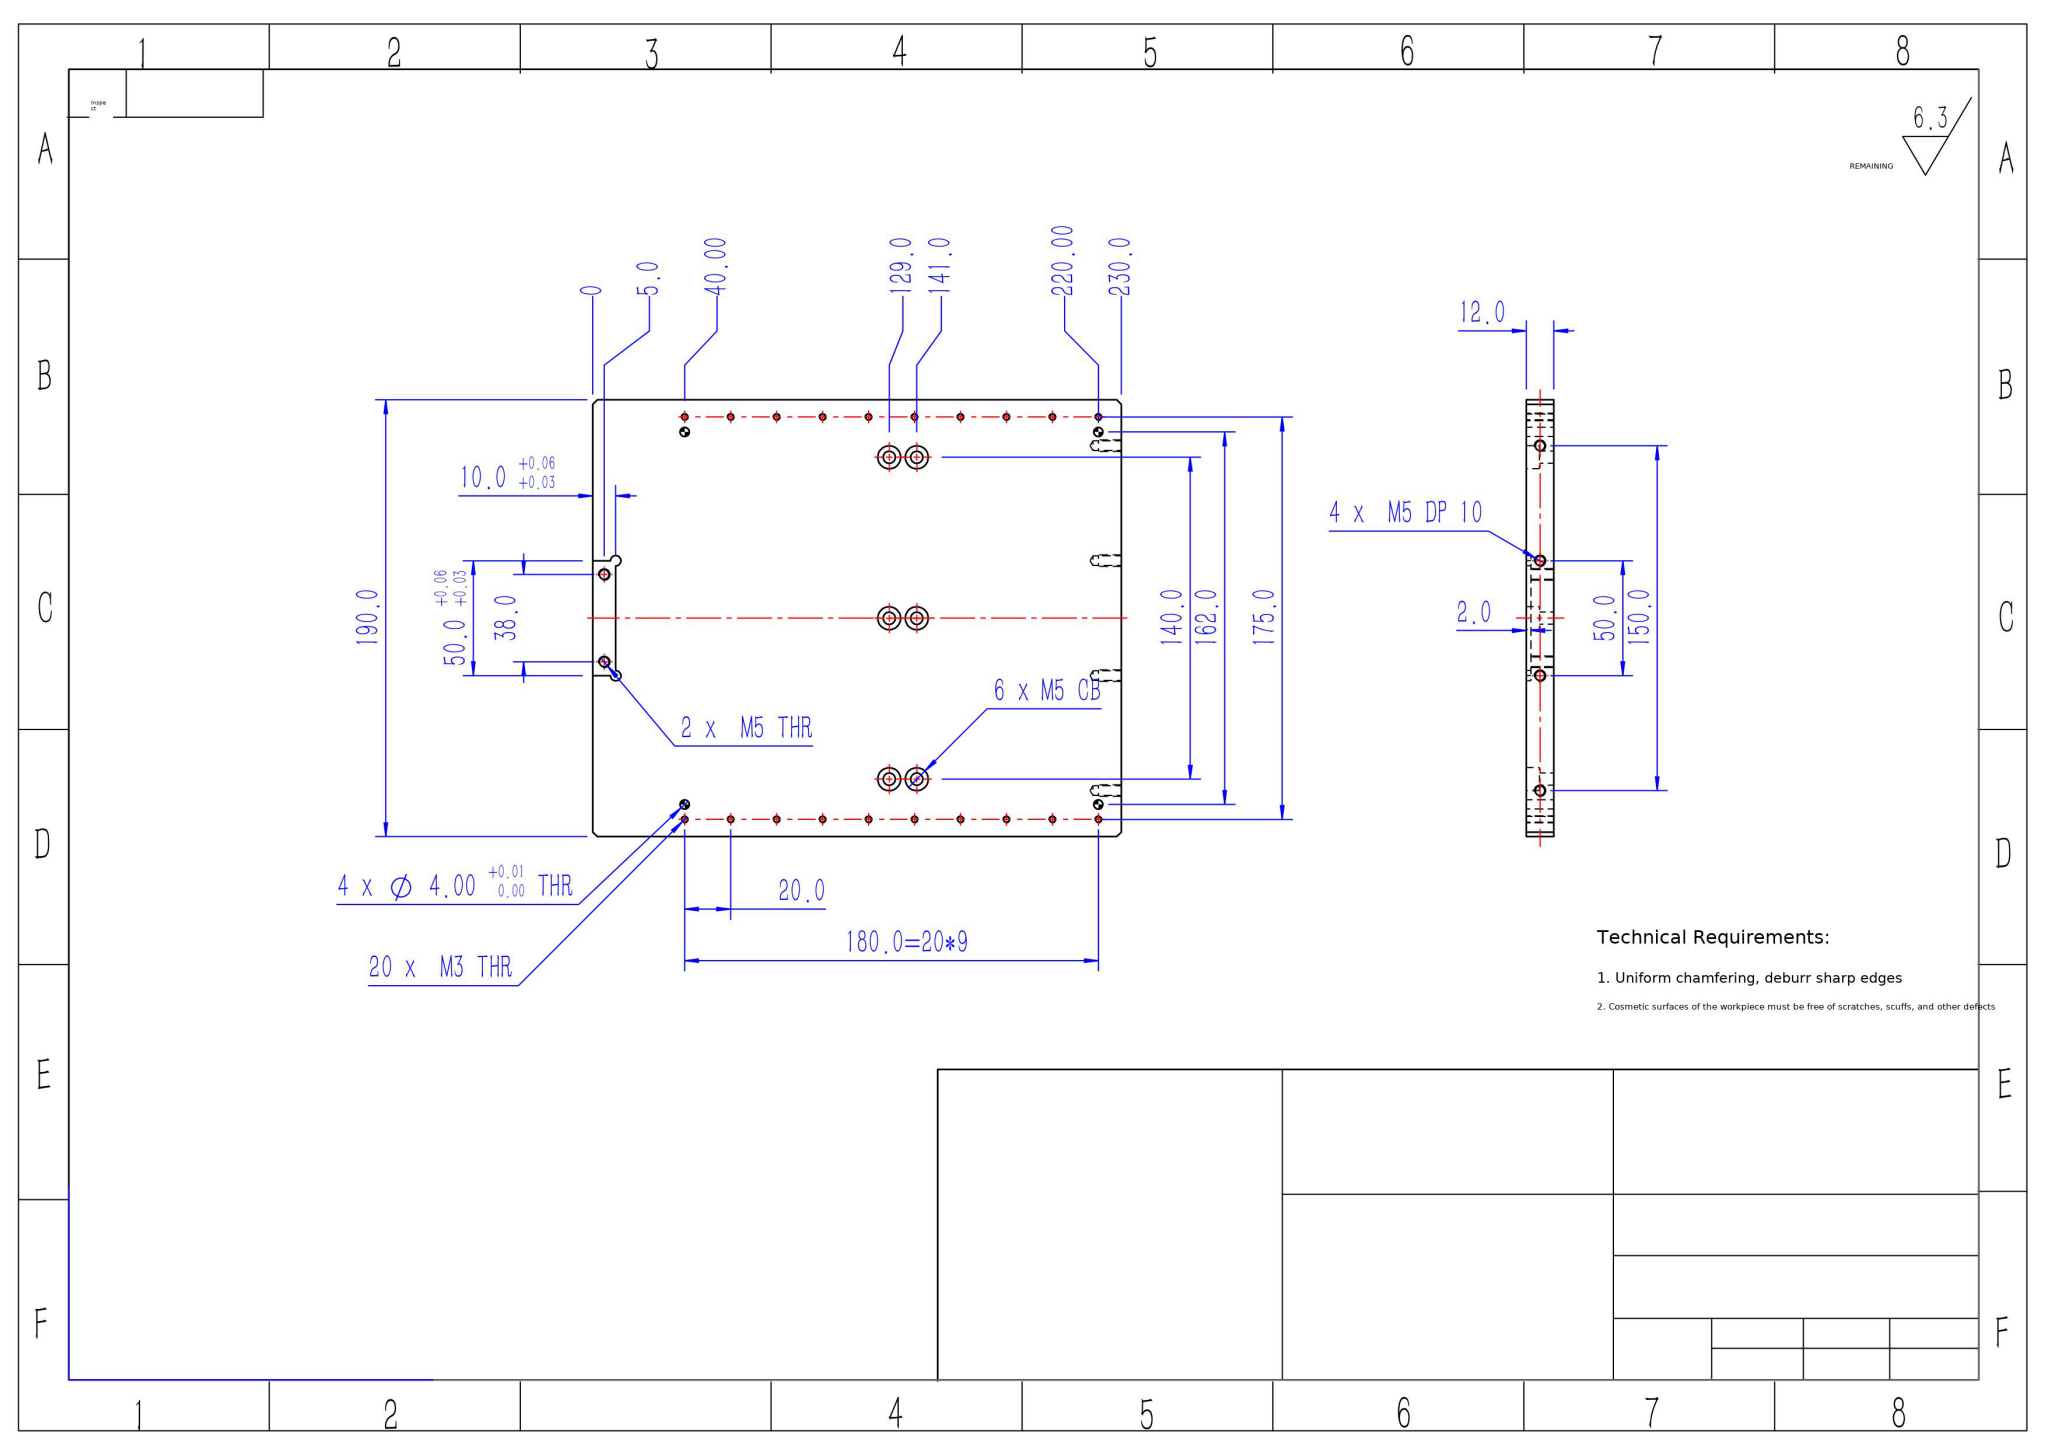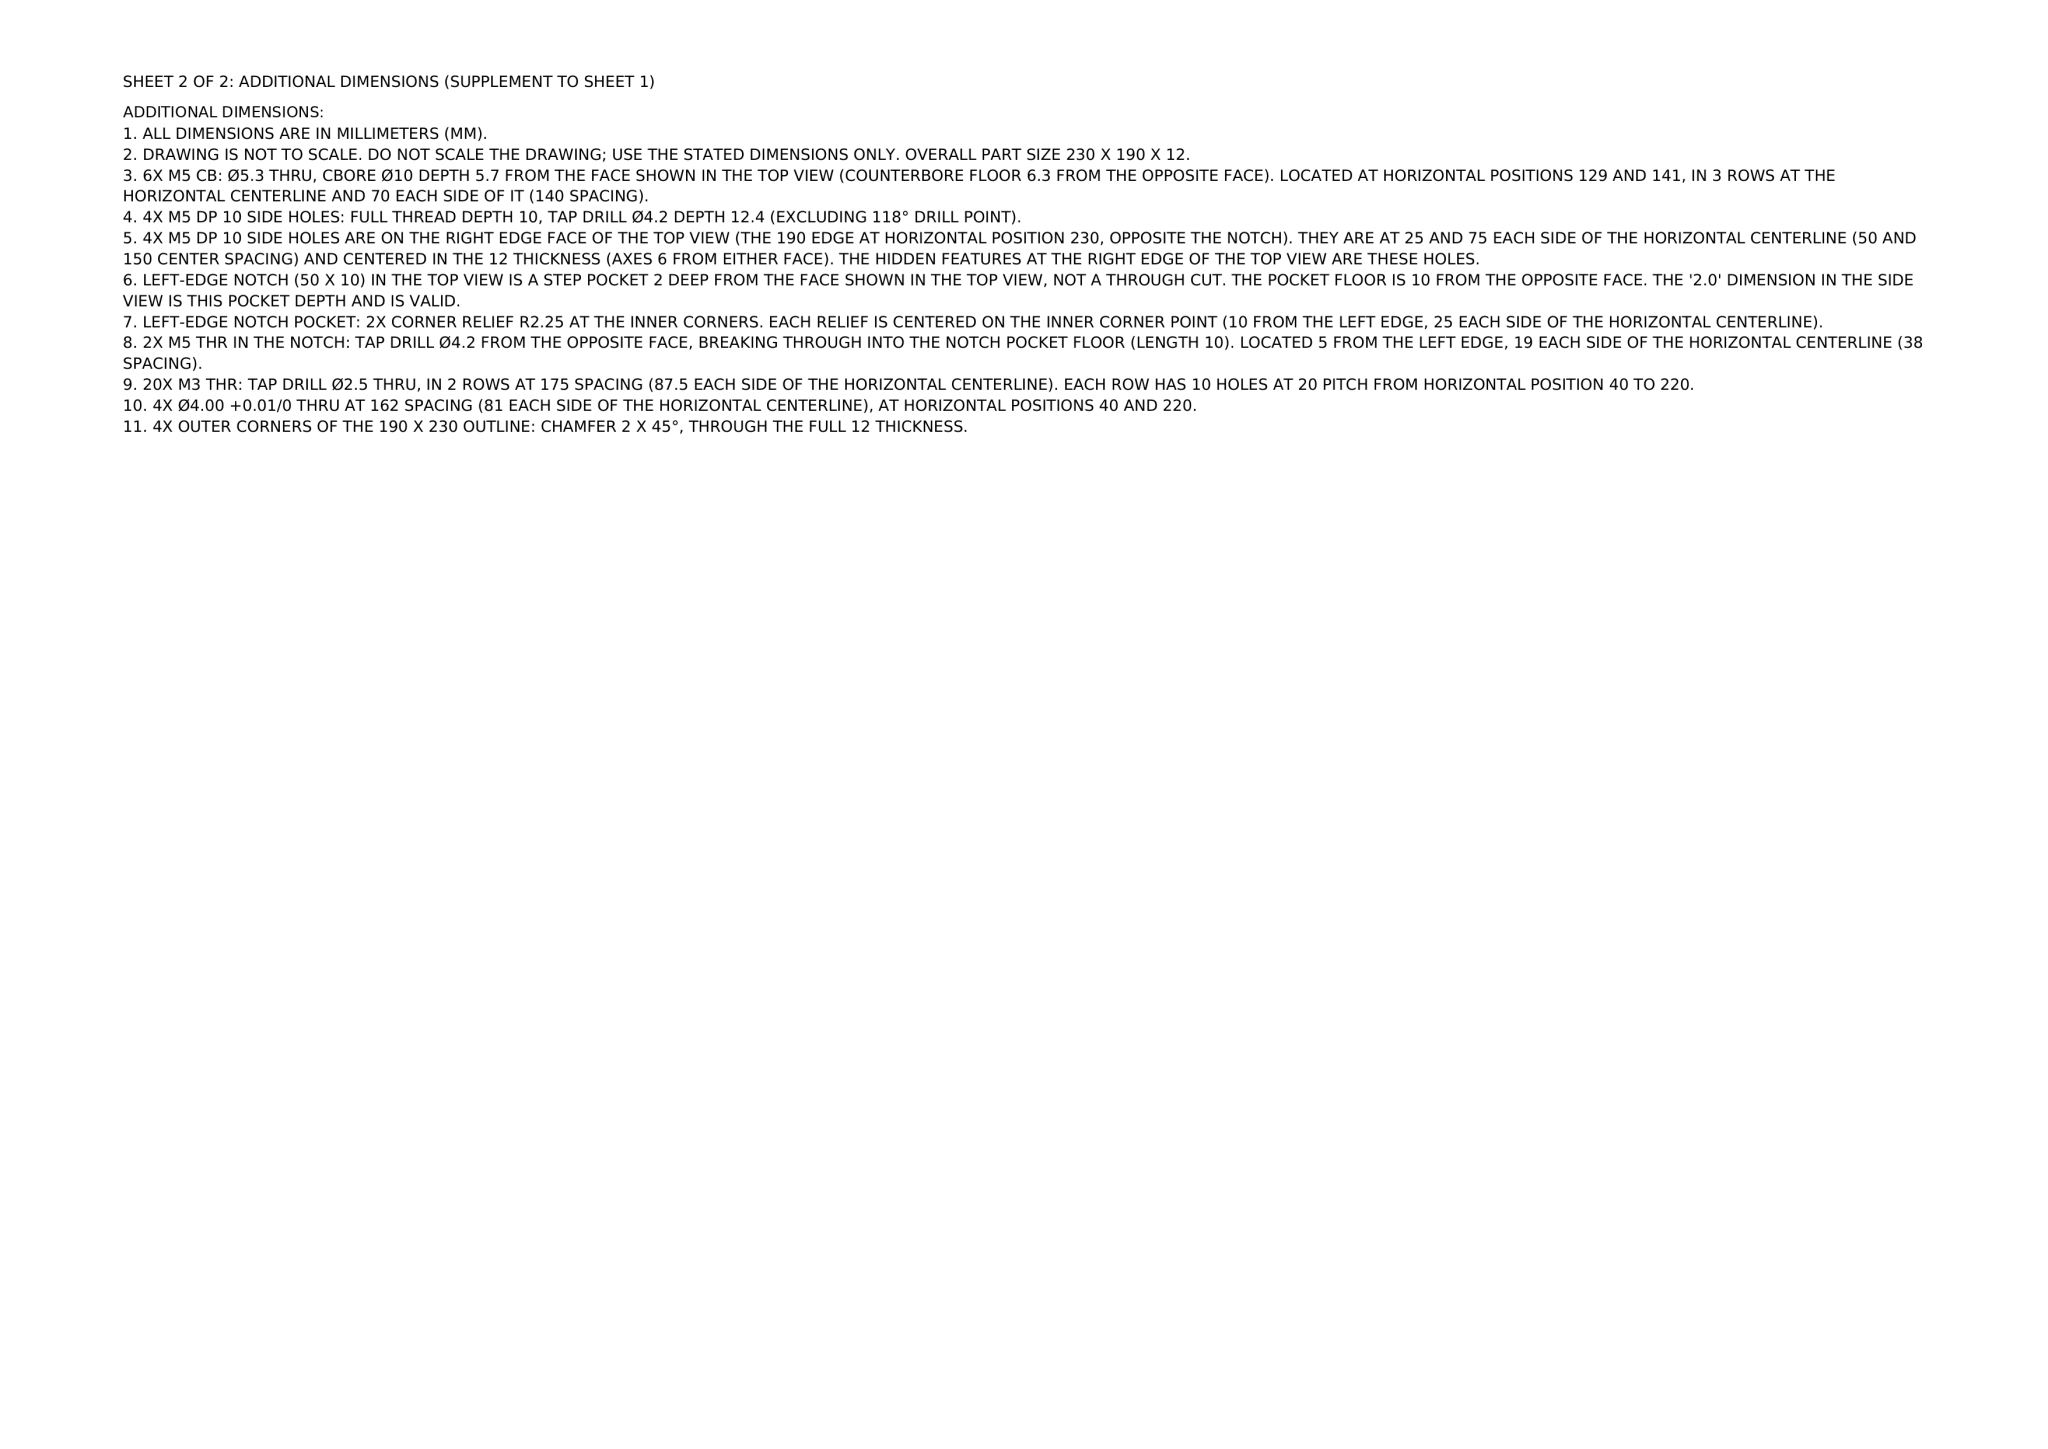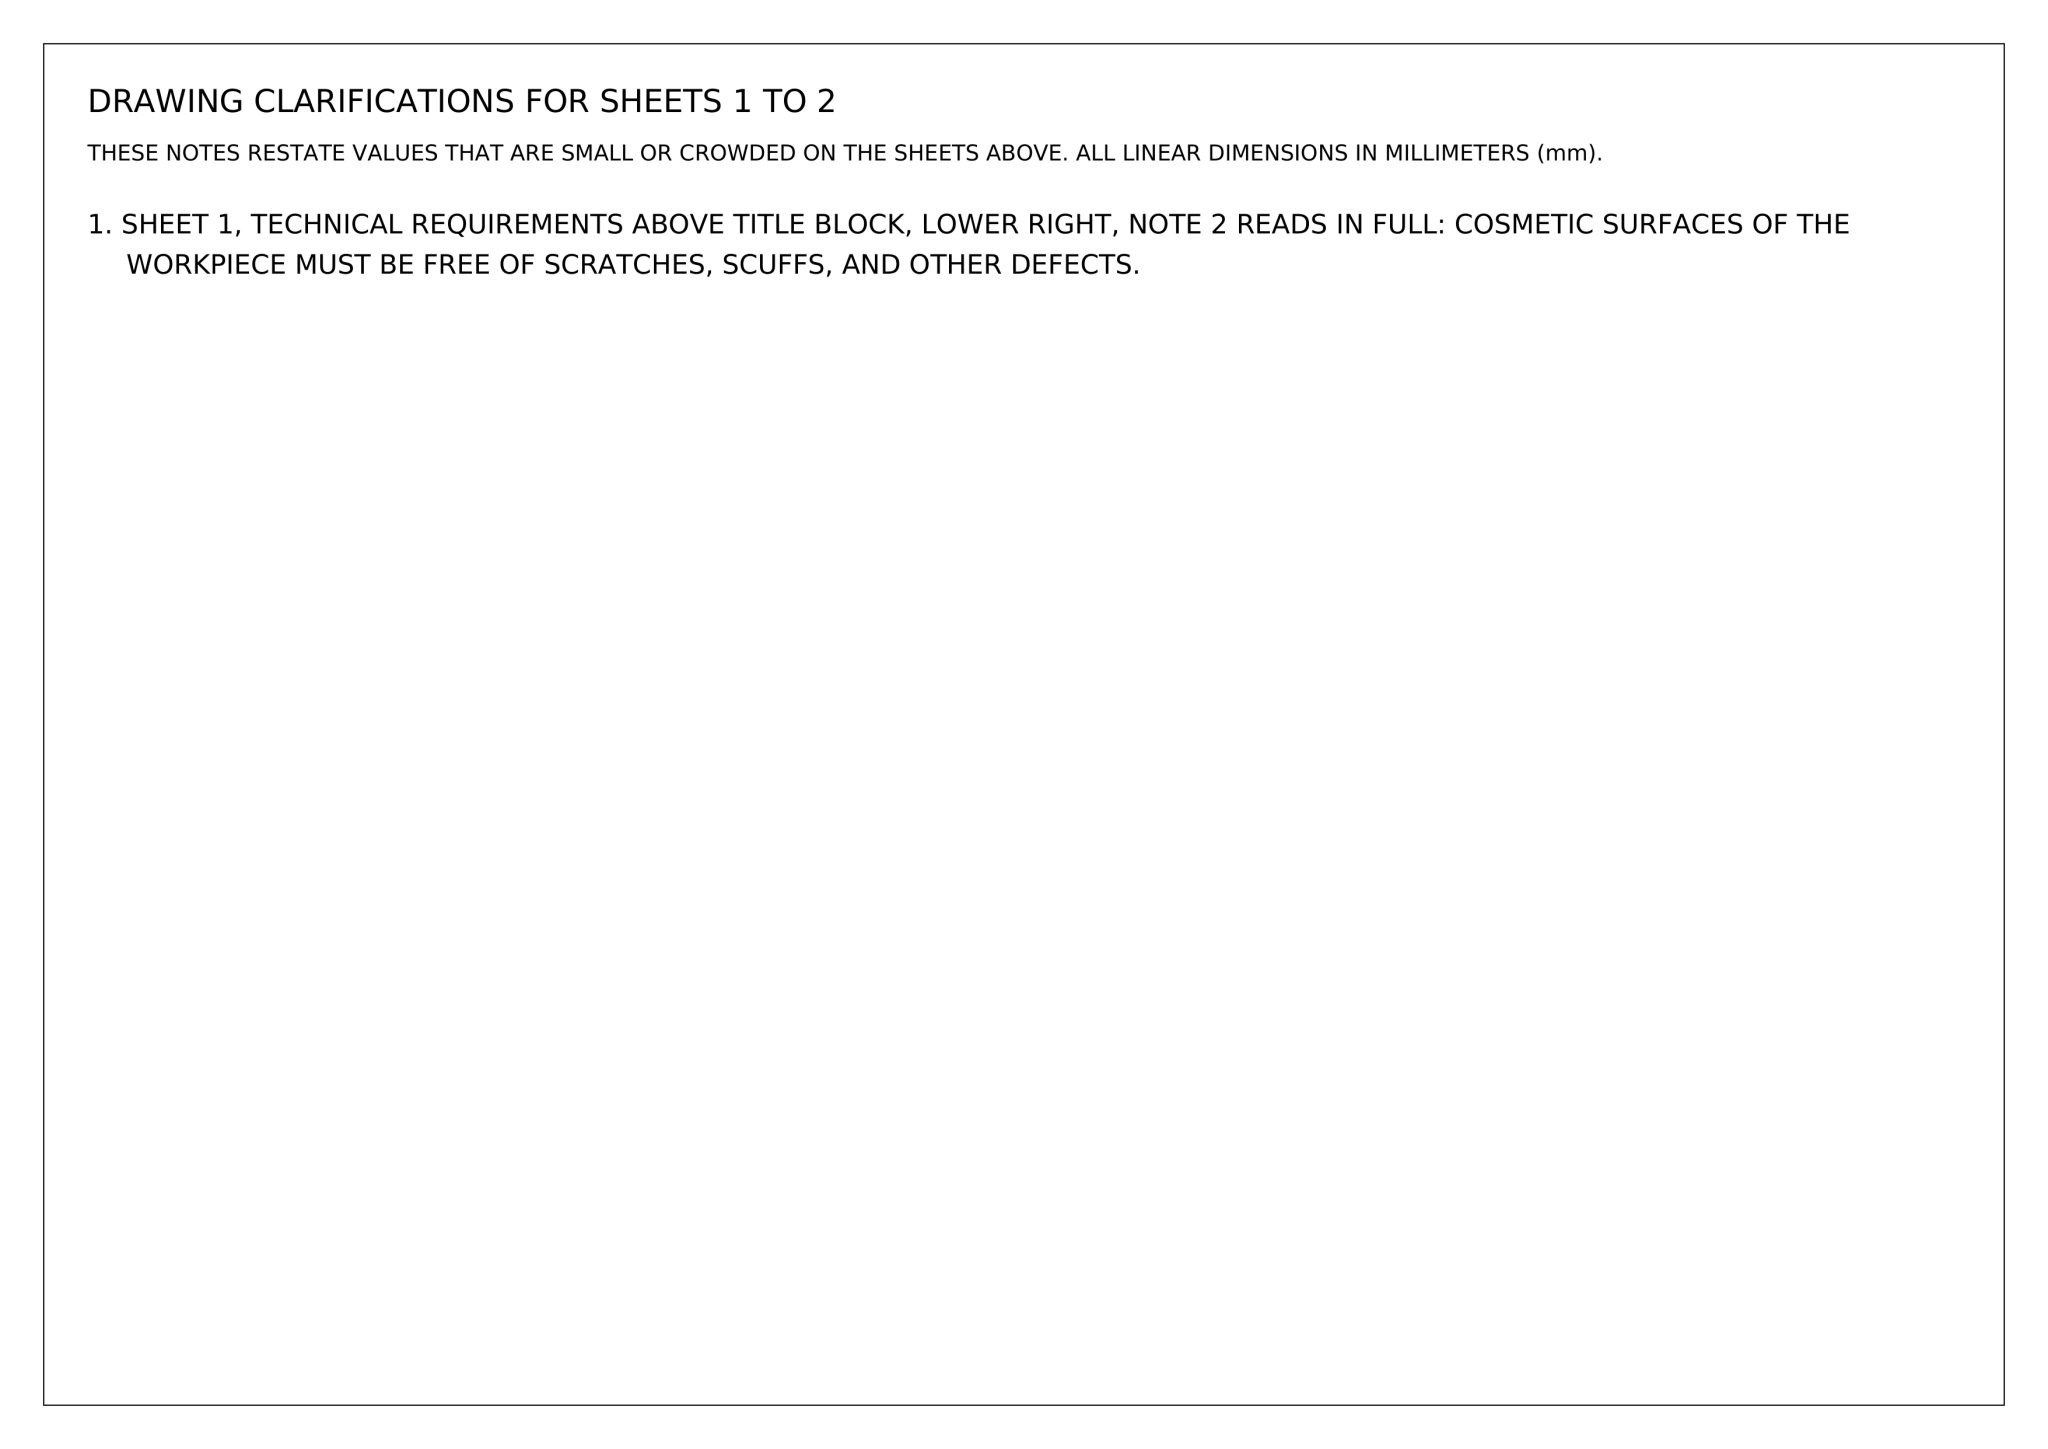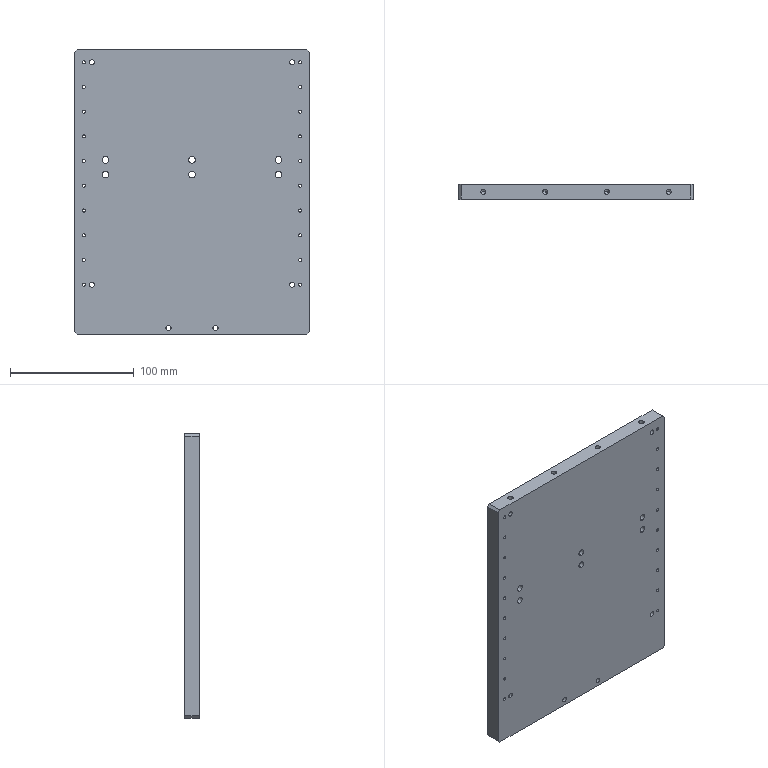Part | NX | mm | 1 solid | 116 faces | box 190 x 12 x 230 mm | volume 516967 mm3 | cylinder 88 | plane 20 | cone 8 | commonest cylinder face diameters 2.5 x40 4.2 x12 10 x12 5.3 x12 4 x8 4.5 x4